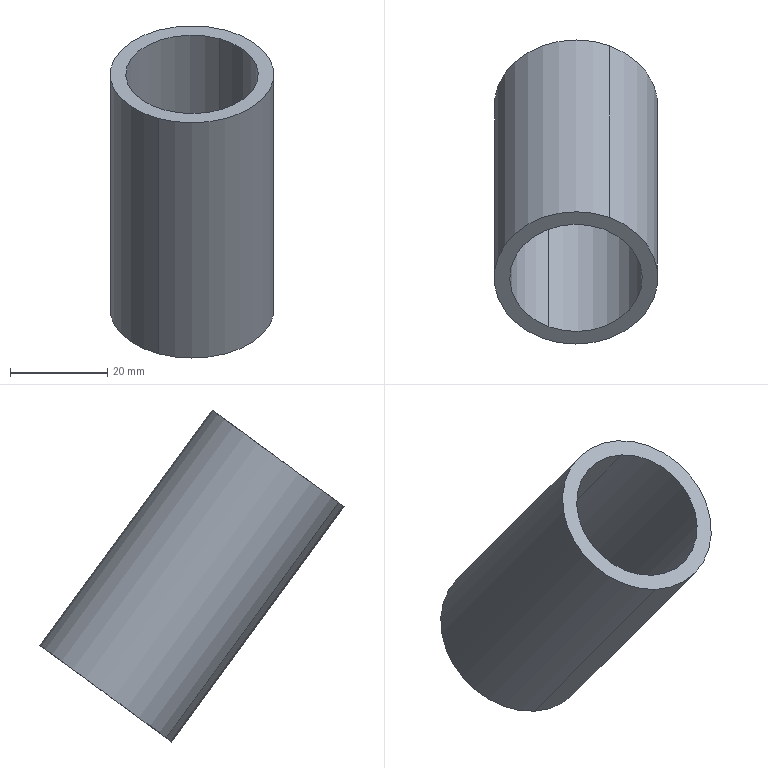Component | SolidWorks | circular tube_iso-1 | 1 solid | 6 faces | box 33.7 x 62.64 x 68.32 mm | volume 18397 mm3 | cylinder 4 | plane 2 | commonest cylinder face diameters 27.3 x2 33.7 x2
STEP:
#1=COLOUR_RGB('',0.7922,0.8196,0.9333);
#2=FILL_AREA_STYLE_COLOUR('',#1);
#3=FILL_AREA_STYLE('',(#2));
#4=SURFACE_STYLE_FILL_AREA(#3);
#5=SURFACE_SIDE_STYLE('',(#4));
#6=SURFACE_STYLE_USAGE(.BOTH.,#5);
#7=PRESENTATION_STYLE_ASSIGNMENT((#6));
#8=CARTESIAN_POINT('',(-11.187,27.132,10.421));
#9=VERTEX_POINT('',#8);
#10=CARTESIAN_POINT('',(-10.75,27.924,11.001));
#11=VERTEX_POINT('',#10);
#12=CARTESIAN_POINT('',(-10.969,27.528,10.711));
#13=DIRECTION('',(0.,-0.5907,0.8069));
#14=DIRECTION('',(0.4071,0.737,0.5396));
#15=AXIS2_PLACEMENT_3D('',#12,#13,#14);
#16=CIRCLE('',#15,0.5374);
#17=EDGE_CURVE('',#9,#11,#16,.T.);
#18=ORIENTED_EDGE('',*,*,#17,.T.);
#19=CARTESIAN_POINT('',(-10.75,29.319,9.095));
#20=VERTEX_POINT('',#19);
#21=CARTESIAN_POINT('',(-10.75,27.924,11.001));
#22=DIRECTION('',(0.,0.5907,-0.8069));
#23=VECTOR('',#22,39.37);
#24=LINE('',#21,#23);
#25=EDGE_CURVE('',#11,#20,#24,.T.);
#26=ORIENTED_EDGE('',*,*,#25,.T.);
#27=CARTESIAN_POINT('',(-11.187,28.527,8.515));
#28=VERTEX_POINT('',#27);
#29=CARTESIAN_POINT('',(-10.969,28.923,8.805));
#30=DIRECTION('',(0.,-0.5907,0.8069));
#31=DIRECTION('',(0.4071,0.737,0.5396));
#32=AXIS2_PLACEMENT_3D('',#29,#30,#31);
#33=CIRCLE('',#32,0.5374);
#34=EDGE_CURVE('',#28,#20,#33,.T.);
#35=ORIENTED_EDGE('',*,*,#34,.F.);
#36=CARTESIAN_POINT('',(-11.187,27.132,10.421));
#37=DIRECTION('',(0.,0.5907,-0.8069));
#38=VECTOR('',#37,39.37);
#39=LINE('',#36,#38);
#40=EDGE_CURVE('',#9,#28,#39,.T.);
#41=ORIENTED_EDGE('',*,*,#40,.F.);
#42=EDGE_LOOP('',(#18,#26,#35,#41));
#43=FACE_OUTER_BOUND('',#42,.T.);
#44=CARTESIAN_POINT('',(-10.969,27.528,10.711));
#45=DIRECTION('',(0.,0.5907,-0.8069));
#46=DIRECTION('',(-0.4071,-0.737,-0.5396));
#47=AXIS2_PLACEMENT_3D('',#44,#45,#46);
#48=CYLINDRICAL_SURFACE('',#47,0.5374);
#49=ADVANCED_FACE('',(#43),#48,.F.);
#50=CARTESIAN_POINT('',(-10.698,28.017,11.069));
#51=VERTEX_POINT('',#50);
#52=CARTESIAN_POINT('',(-11.239,27.039,10.353));
#53=VERTEX_POINT('',#52);
#54=CARTESIAN_POINT('',(-10.969,27.528,10.711));
#55=DIRECTION('',(0.,-0.5907,0.8069));
#56=DIRECTION('',(0.4071,0.737,0.5396));
#57=AXIS2_PLACEMENT_3D('',#54,#55,#56);
#58=CIRCLE('',#57,0.6634);
#59=EDGE_CURVE('',#51,#53,#58,.T.);
#60=ORIENTED_EDGE('',*,*,#59,.F.);
#61=CARTESIAN_POINT('',(-10.698,29.412,9.163));
#62=VERTEX_POINT('',#61);
#63=CARTESIAN_POINT('',(-10.698,28.017,11.069));
#64=DIRECTION('',(0.,0.5907,-0.8069));
#65=VECTOR('',#64,39.37);
#66=LINE('',#63,#65);
#67=EDGE_CURVE('',#51,#62,#66,.T.);
#68=ORIENTED_EDGE('',*,*,#67,.T.);
#69=CARTESIAN_POINT('',(-11.239,28.434,8.447));
#70=VERTEX_POINT('',#69);
#71=CARTESIAN_POINT('',(-10.969,28.923,8.805));
#72=DIRECTION('',(0.,-0.5907,0.8069));
#73=DIRECTION('',(0.4071,0.737,0.5396));
#74=AXIS2_PLACEMENT_3D('',#71,#72,#73);
#75=CIRCLE('',#74,0.6634);
#76=EDGE_CURVE('',#62,#70,#75,.T.);
#77=ORIENTED_EDGE('',*,*,#76,.T.);
#78=CARTESIAN_POINT('',(-11.239,27.039,10.353));
#79=DIRECTION('',(0.,0.5907,-0.8069));
#80=VECTOR('',#79,39.37);
#81=LINE('',#78,#80);
#82=EDGE_CURVE('',#53,#70,#81,.T.);
#83=ORIENTED_EDGE('',*,*,#82,.F.);
#84=EDGE_LOOP('',(#60,#68,#77,#83));
#85=FACE_OUTER_BOUND('',#84,.T.);
#86=CARTESIAN_POINT('',(-10.969,27.528,10.711));
#87=DIRECTION('',(0.,0.5907,-0.8069));
#88=DIRECTION('',(-0.4071,-0.737,-0.5396));
#89=AXIS2_PLACEMENT_3D('',#86,#87,#88);
#90=CYLINDRICAL_SURFACE('',#89,0.6634);
#91=ADVANCED_FACE('',(#85),#90,.T.);
#92=CARTESIAN_POINT('',(-10.969,27.528,10.711));
#93=DIRECTION('',(0.,-0.5907,0.8069));
#94=DIRECTION('',(0.4071,0.737,0.5396));
#95=AXIS2_PLACEMENT_3D('',#92,#93,#94);
#96=CIRCLE('',#95,0.6634);
#97=EDGE_CURVE('',#53,#51,#96,.T.);
#98=ORIENTED_EDGE('',*,*,#97,.T.);
#99=ORIENTED_EDGE('',*,*,#59,.T.);
#100=EDGE_LOOP('',(#98,#99));
#101=FACE_OUTER_BOUND('',#100,.T.);
#102=ORIENTED_EDGE('',*,*,#17,.F.);
#103=CARTESIAN_POINT('',(-10.969,27.528,10.711));
#104=DIRECTION('',(0.,-0.5907,0.8069));
#105=DIRECTION('',(0.4071,0.737,0.5396));
#106=AXIS2_PLACEMENT_3D('',#103,#104,#105);
#107=CIRCLE('',#106,0.5374);
#108=EDGE_CURVE('',#11,#9,#107,.T.);
#109=ORIENTED_EDGE('',*,*,#108,.F.);
#110=EDGE_LOOP('',(#102,#109));
#111=FACE_BOUND('',#110,.T.);
#112=CARTESIAN_POINT('',(-10.969,27.528,10.711));
#113=DIRECTION('',(0.,-0.5907,0.8069));
#114=DIRECTION('',(0.4071,0.737,0.5396));
#115=AXIS2_PLACEMENT_3D('',#112,#113,#114);
#116=PLANE('',#115);
#117=ADVANCED_FACE('',(#101,#111),#116,.T.);
#118=CARTESIAN_POINT('',(-10.969,28.923,8.805));
#119=DIRECTION('',(0.,-0.5907,0.8069));
#120=DIRECTION('',(0.4071,0.737,0.5396));
#121=AXIS2_PLACEMENT_3D('',#118,#119,#120);
#122=CIRCLE('',#121,0.6634);
#123=EDGE_CURVE('',#70,#62,#122,.T.);
#124=ORIENTED_EDGE('',*,*,#123,.F.);
#125=ORIENTED_EDGE('',*,*,#76,.F.);
#126=EDGE_LOOP('',(#124,#125));
#127=FACE_OUTER_BOUND('',#126,.T.);
#128=ORIENTED_EDGE('',*,*,#34,.T.);
#129=CARTESIAN_POINT('',(-10.969,28.923,8.805));
#130=DIRECTION('',(0.,-0.5907,0.8069));
#131=DIRECTION('',(0.4071,0.737,0.5396));
#132=AXIS2_PLACEMENT_3D('',#129,#130,#131);
#133=CIRCLE('',#132,0.5374);
#134=EDGE_CURVE('',#20,#28,#133,.T.);
#135=ORIENTED_EDGE('',*,*,#134,.T.);
#136=EDGE_LOOP('',(#128,#135));
#137=FACE_BOUND('',#136,.T.);
#138=CARTESIAN_POINT('',(-10.969,28.923,8.805));
#139=DIRECTION('',(0.,-0.5907,0.8069));
#140=DIRECTION('',(0.4071,0.737,0.5396));
#141=AXIS2_PLACEMENT_3D('',#138,#139,#140);
#142=PLANE('',#141);
#143=ADVANCED_FACE('',(#127,#137),#142,.F.);
#144=ORIENTED_EDGE('',*,*,#67,.F.);
#145=ORIENTED_EDGE('',*,*,#97,.F.);
#146=ORIENTED_EDGE('',*,*,#82,.T.);
#147=ORIENTED_EDGE('',*,*,#123,.T.);
#148=EDGE_LOOP('',(#144,#145,#146,#147));
#149=FACE_OUTER_BOUND('',#148,.T.);
#150=CARTESIAN_POINT('',(-10.969,27.528,10.711));
#151=DIRECTION('',(0.,0.5907,-0.8069));
#152=DIRECTION('',(-0.4071,-0.737,-0.5396));
#153=AXIS2_PLACEMENT_3D('',#150,#151,#152);
#154=CYLINDRICAL_SURFACE('',#153,0.6634);
#155=ADVANCED_FACE('',(#149),#154,.T.);
#156=ORIENTED_EDGE('',*,*,#25,.F.);
#157=ORIENTED_EDGE('',*,*,#108,.T.);
#158=ORIENTED_EDGE('',*,*,#40,.T.);
#159=ORIENTED_EDGE('',*,*,#134,.F.);
#160=EDGE_LOOP('',(#156,#157,#158,#159));
#161=FACE_OUTER_BOUND('',#160,.T.);
#162=CARTESIAN_POINT('',(-10.969,27.528,10.711));
#163=DIRECTION('',(0.,0.5907,-0.8069));
#164=DIRECTION('',(-0.4071,-0.737,-0.5396));
#165=AXIS2_PLACEMENT_3D('',#162,#163,#164);
#166=CYLINDRICAL_SURFACE('',#165,0.5374);
#167=ADVANCED_FACE('',(#161),#166,.F.);
#168=CLOSED_SHELL('',(#49,#91,#117,#143,#155,#167));
#169=MANIFOLD_SOLID_BREP('',#168);
#170=STYLED_ITEM('',(#7),#169);
#171=(LENGTH_UNIT()NAMED_UNIT(*)SI_UNIT($,.METRE.));
#172=LENGTH_MEASURE_WITH_UNIT(LENGTH_MEASURE(0.0254),#171);
#173=DIMENSIONAL_EXPONENTS(1.,0.,0.,0.,0.,0.,0.);
#174=(CONVERSION_BASED_UNIT('',#172)LENGTH_UNIT()NAMED_UNIT(#173));
#175=UNCERTAINTY_MEASURE_WITH_UNIT(LENGTH_MEASURE(0.00001),#174,'','');
#176=(NAMED_UNIT(*)PLANE_ANGLE_UNIT()SI_UNIT($,.RADIAN.));
#177=(NAMED_UNIT(*)SI_UNIT($,.STERADIAN.)SOLID_ANGLE_UNIT());
#178=(GEOMETRIC_REPRESENTATION_CONTEXT(3)GLOBAL_UNCERTAINTY_ASSIGNED_CONTEXT((#175))GLOBAL_UNIT_ASSIGNED_CONTEXT((#174,#176,#177))REPRESENTATION_CONTEXT('',''));
#179=MECHANICAL_DESIGN_GEOMETRIC_PRESENTATION_REPRESENTATION('',(#170),#178);
#180=CARTESIAN_POINT('',(0.,0.,0.));
#181=DIRECTION('',(0.,0.,1.));
#182=DIRECTION('',(1.,0.,0.));
#183=AXIS2_PLACEMENT_3D('',#180,#181,#182);
#184=(LENGTH_UNIT()NAMED_UNIT(*)SI_UNIT($,.METRE.));
#185=LENGTH_MEASURE_WITH_UNIT(LENGTH_MEASURE(0.0254),#184);
#186=DIMENSIONAL_EXPONENTS(1.,0.,0.,0.,0.,0.,0.);
#187=(CONVERSION_BASED_UNIT('',#185)LENGTH_UNIT()NAMED_UNIT(#186));
#188=UNCERTAINTY_MEASURE_WITH_UNIT(LENGTH_MEASURE(0.00001),#187,'','');
#189=(NAMED_UNIT(*)PLANE_ANGLE_UNIT()SI_UNIT($,.RADIAN.));
#190=(NAMED_UNIT(*)SI_UNIT($,.STERADIAN.)SOLID_ANGLE_UNIT());
#191=(GEOMETRIC_REPRESENTATION_CONTEXT(3)GLOBAL_UNCERTAINTY_ASSIGNED_CONTEXT((#188))GLOBAL_UNIT_ASSIGNED_CONTEXT((#187,#189,#190))REPRESENTATION_CONTEXT('',''));
#192=ADVANCED_BREP_SHAPE_REPRESENTATION('',(#169,#183),#191);
#193=PRESENTATION_LAYER_ASSIGNMENT('','',(#170));